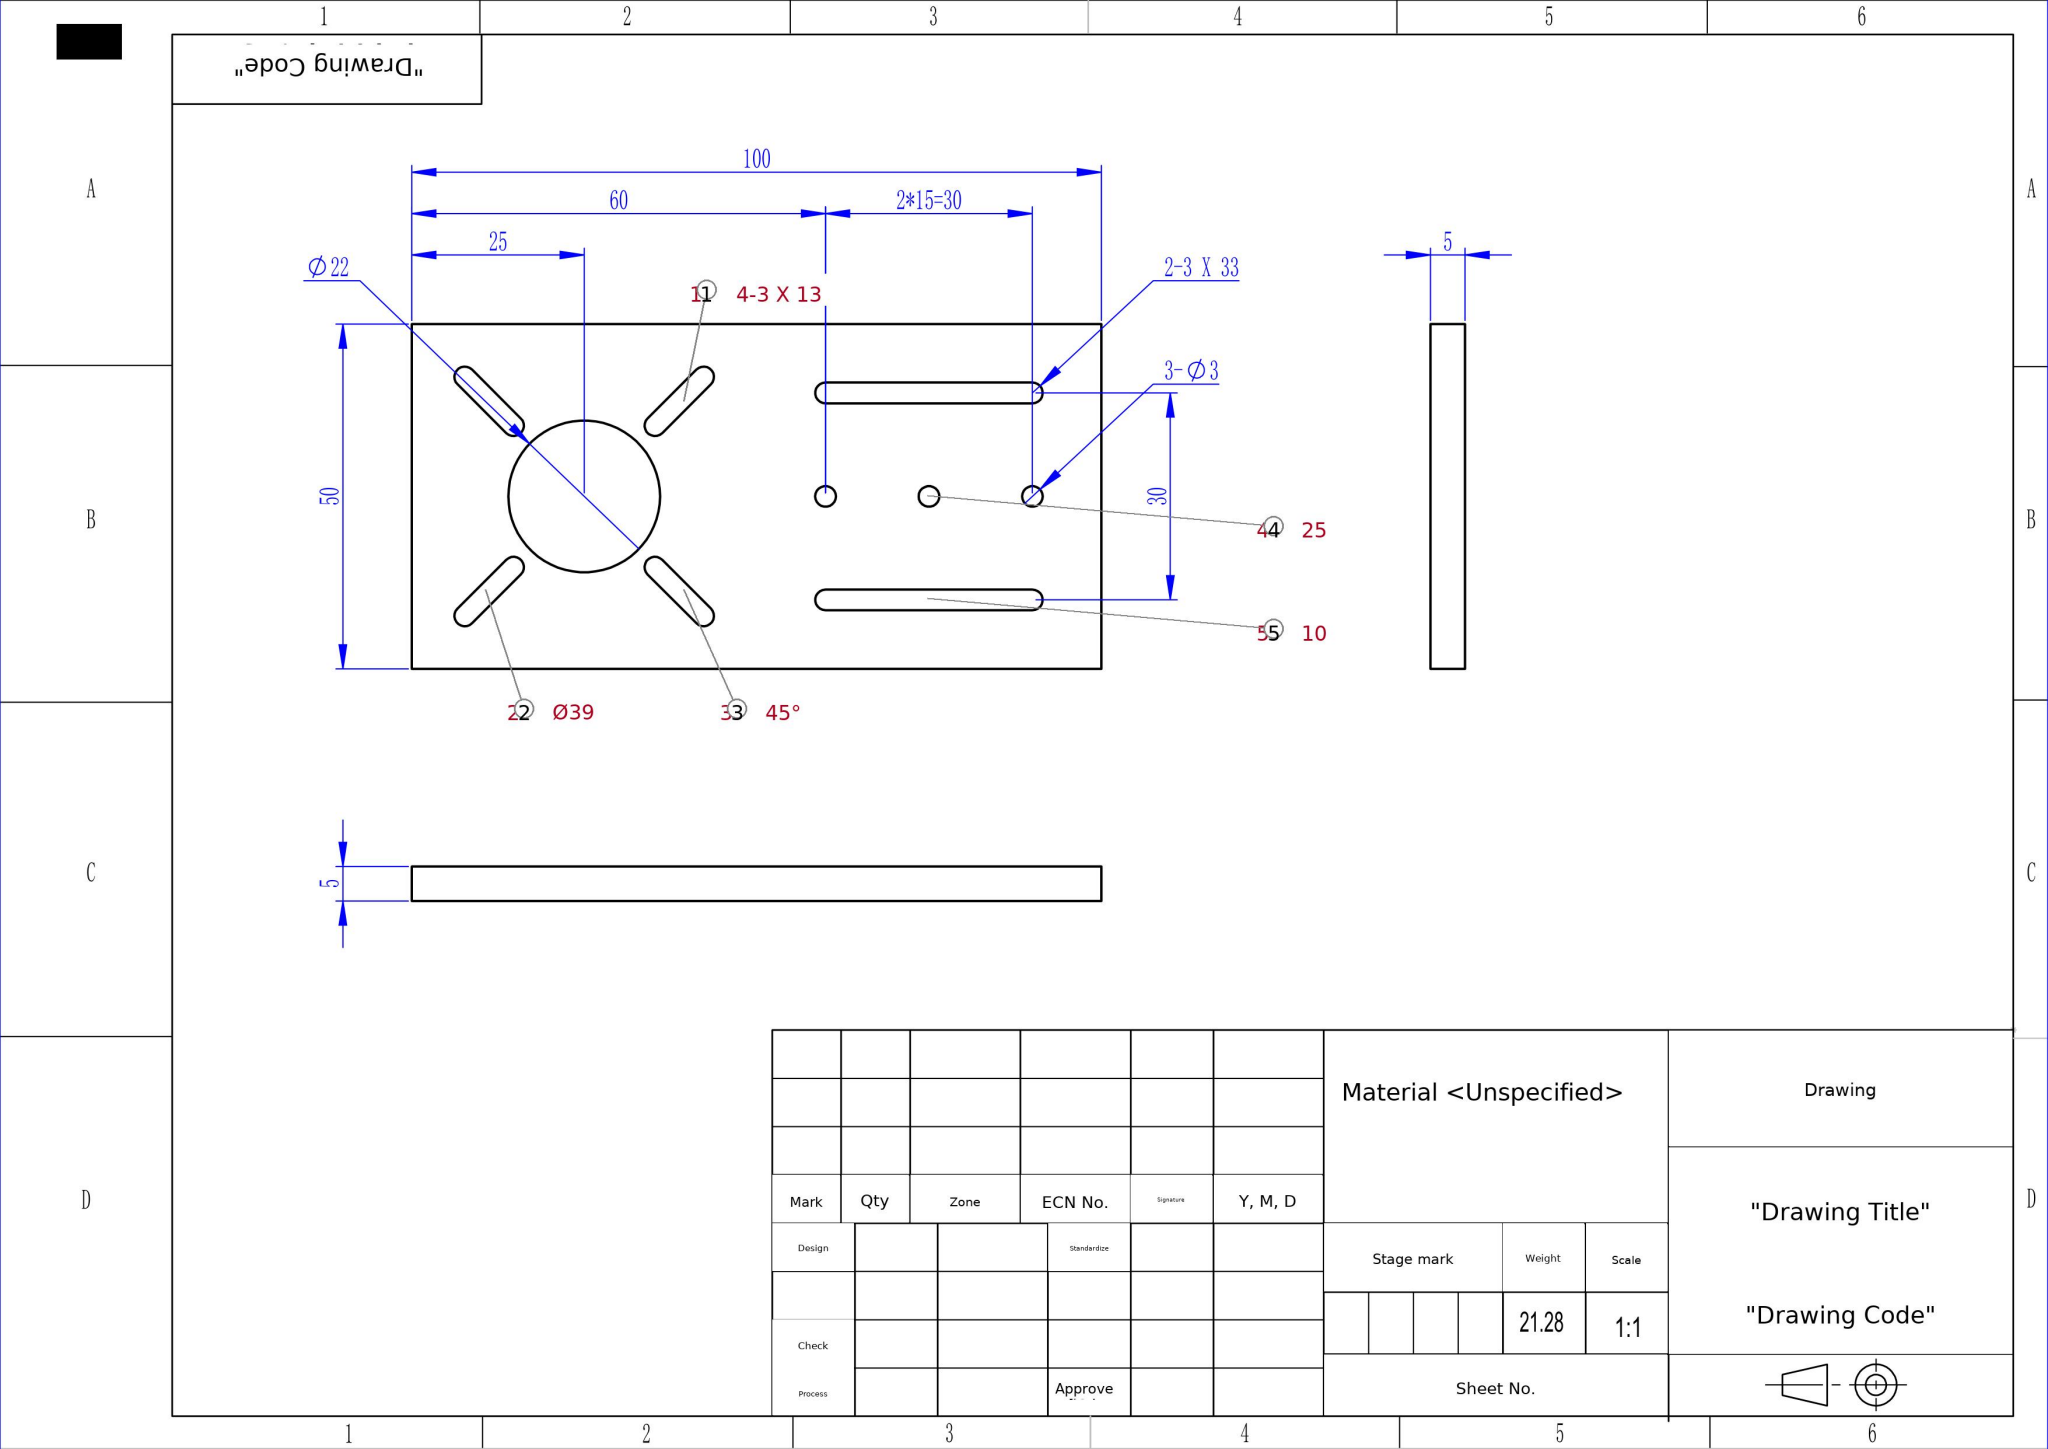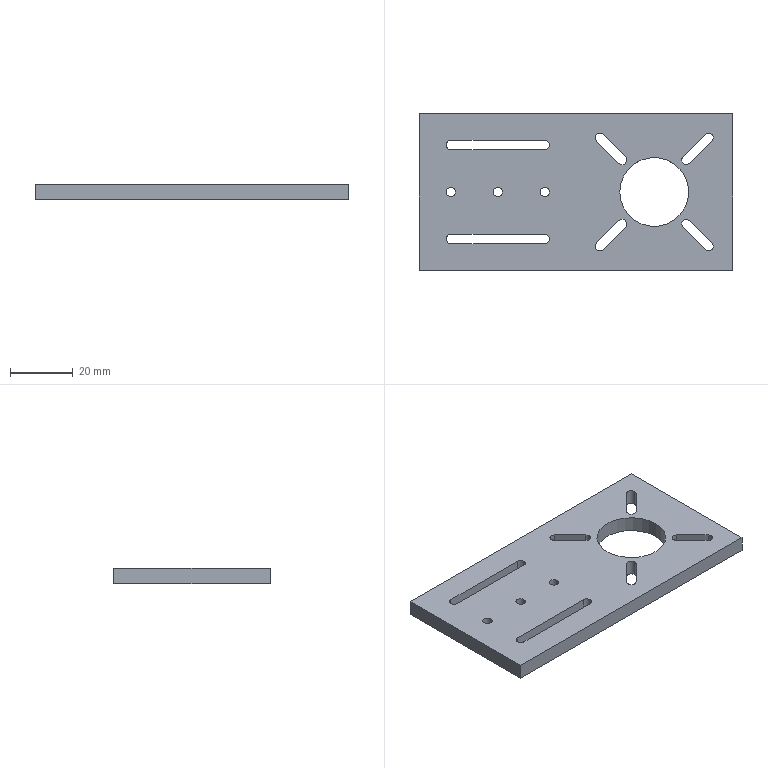Part | SolidWorks | mm | 1 solid | 44 faces | box 100 x 50 x 5 mm | volume 21281 mm3 | cylinder 26 | plane 18 | commonest cylinder face diameters 3 x24 22 x2
build123d program:
from build123d import *

# Parameters (mm, degrees)
BOSS_EXTRUDE1_DEPTH = 5


with BuildPart() as part:
    # Sketch1 → Boss-Extrude1 (new body)
    # profile 1 of 11: a face of its own
    with BuildSketch(Plane.XY):
        with BuildLine():
            Line((-8.5, 0), (0, 0))
            Line((0, 0), (0, 25))
            Line((0, 25), (-41.5, 25))
            Line((-41.5, 25), (-41.5, 15))
            Line((-41.5, 15), (-41.5, 0))
            ThreePointArc((-41.5, 0), (-40, 1.5), (-38.5, 0))
            Line((-38.5, 0), (-26.5, 0))
            ThreePointArc((-26.5, 0), (-25, 1.5), (-23.5, 0))
            Line((-23.5, 0), (-11.5, 0))
            ThreePointArc((-11.5, 0), (-10, 1.5), (-8.5, 0))
        make_face()
        with BuildLine():
            ThreePointArc((-40, 13.5), (-41.061, 13.939), (-41.5, 15))
            ThreePointArc((-41.5, 15), (-41.061, 16.061), (-40, 16.5))
            Line((-40, 16.5), (-10, 16.5))
            ThreePointArc((-10, 16.5), (-8.5, 15), (-10, 13.5))
            Line((-10, 13.5), (-40, 13.5))
        make_face(mode=Mode.SUBTRACT)
    # profile 2 of 11: a face of its own
    with BuildSketch(Plane.XY):
        Polygon((-41.5, 15), (-41.5, 25), (-50, 25), (-50, 0), (-41.5, 0), align=None)
    # profile 3 of 11: a face of its own
    with BuildSketch(Plane.XY):
        with BuildLine():
            Line((0, -25), (0, 0))
            Line((0, 0), (-8.5, 0))
            ThreePointArc((-8.5, 0), (-10, -1.5), (-11.5, 0))
            Line((-11.5, 0), (-23.5, 0))
            ThreePointArc((-23.5, 0), (-25, -1.5), (-26.5, 0))
            Line((-26.5, 0), (-38.5, 0))
            ThreePointArc((-38.5, 0), (-40, -1.5), (-41.5, 0))
            Line((-41.5, 0), (-50, 0))
            Line((-50, 0), (-50, -25))
            Line((-50, -25), (0, -25))
        make_face()
        with BuildLine():
            Line((-10, -16.5), (-40, -16.5))
            ThreePointArc((-40, -16.5), (-41.5, -15), (-40, -13.5))
            Line((-40, -13.5), (-10, -13.5))
            ThreePointArc((-10, -13.5), (-8.5, -15), (-10, -16.5))
        make_face(mode=Mode.SUBTRACT)
    # profile 4 of 11: a face of its own
    with BuildSketch(Plane.XY):
        with BuildLine():
            Line((0, 0), (14, 0))
            ThreePointArc((14, 0), (14.837, 4.21), (17.222, 7.778))
            Line((17.222, 7.778), (15.808, 9.192))
            ThreePointArc((15.808, 9.192), (14.747, 8.753), (13.686, 9.192))
            Line((13.686, 9.192), (6.615, 16.263))
            ThreePointArc((6.615, 16.263), (6.176, 17.324), (6.615, 18.385))
            Line((6.615, 18.385), (0, 25))
            Line((0, 25), (0, 0))
        make_face()
    # profile 5 of 11: a face of its own
    with BuildSketch(Plane.XY):
        with BuildLine():
            Line((15.808, 9.192), (17.222, 7.778))
            ThreePointArc((17.222, 7.778), (20.79, 10.163), (25, 11))
            Line((25, 11), (25, 25))
            Line((25, 25), (0, 25))
            Line((0, 25), (6.615, 18.385))
            ThreePointArc((6.615, 18.385), (7.676, 18.824), (8.737, 18.385))
            Line((8.737, 18.385), (15.808, 11.314))
            ThreePointArc((15.808, 11.314), (16.247, 10.253), (15.808, 9.192))
        make_face()
    # profile 6 of 11: a face of its own
    with BuildSketch(Plane.XY):
        with BuildLine():
            ThreePointArc((25, 11), (29.21, 10.163), (32.778, 7.778))
            Line((32.778, 7.778), (34.192, 9.192))
            ThreePointArc((34.192, 9.192), (33.753, 10.253), (34.192, 11.314))
            Line((34.192, 11.314), (41.263, 18.385))
            ThreePointArc((41.263, 18.385), (42.324, 18.824), (43.385, 18.385))
            Line((43.385, 18.385), (50, 25))
            Line((50, 25), (25, 25))
            Line((25, 25), (25, 11))
        make_face()
    # profile 7 of 11: a face of its own
    with BuildSketch(Plane.XY):
        with BuildLine():
            ThreePointArc((32.778, 7.778), (35.163, 4.21), (36, 0))
            Line((36, 0), (50, 0))
            Line((50, 0), (50, 25))
            Line((50, 25), (43.385, 18.385))
            ThreePointArc((43.385, 18.385), (43.824, 17.324), (43.385, 16.263))
            Line((43.385, 16.263), (36.314, 9.192))
            ThreePointArc((36.314, 9.192), (35.253, 8.753), (34.192, 9.192))
            Line((34.192, 9.192), (32.778, 7.778))
        make_face()
    # profile 8 of 11: a face of its own
    with BuildSketch(Plane.XY):
        with BuildLine():
            Line((50, 0), (36, 0))
            ThreePointArc((36, 0), (35.163, -4.21), (32.778, -7.778))
            Line((32.778, -7.778), (34.192, -9.192))
            ThreePointArc((34.192, -9.192), (35.253, -8.753), (36.314, -9.192))
            Line((36.314, -9.192), (43.385, -16.263))
            ThreePointArc((43.385, -16.263), (43.824, -17.324), (43.385, -18.385))
            Line((43.385, -18.385), (50, -25))
            Line((50, -25), (50, 0))
        make_face()
    # profile 9 of 11: a face of its own
    with BuildSketch(Plane.XY):
        with BuildLine():
            Line((34.192, -9.192), (32.778, -7.778))
            ThreePointArc((32.778, -7.778), (29.21, -10.163), (25, -11))
            Line((25, -11), (25, -25))
            Line((25, -25), (50, -25))
            Line((50, -25), (43.385, -18.385))
            ThreePointArc((43.385, -18.385), (42.324, -18.824), (41.263, -18.385))
            Line((41.263, -18.385), (34.192, -11.314))
            ThreePointArc((34.192, -11.314), (33.753, -10.253), (34.192, -9.192))
        make_face()
    # profile 10 of 11: a face of its own
    with BuildSketch(Plane.XY):
        with BuildLine():
            ThreePointArc((25, -11), (20.79, -10.163), (17.222, -7.778))
            Line((17.222, -7.778), (15.808, -9.192))
            ThreePointArc((15.808, -9.192), (16.247, -10.253), (15.808, -11.314))
            Line((15.808, -11.314), (8.737, -18.385))
            ThreePointArc((8.737, -18.385), (7.676, -18.824), (6.615, -18.385))
            Line((6.615, -18.385), (0, -25))
            Line((0, -25), (25, -25))
            Line((25, -25), (25, -11))
        make_face()
    # profile 11 of 11: a face of its own
    with BuildSketch(Plane.XY):
        with BuildLine():
            ThreePointArc((17.222, -7.778), (14.837, -4.21), (14, 0))
            Line((14, 0), (0, 0))
            Line((0, 0), (0, -25))
            Line((0, -25), (6.615, -18.385))
            ThreePointArc((6.615, -18.385), (6.176, -17.324), (6.615, -16.263))
            Line((6.615, -16.263), (13.686, -9.192))
            ThreePointArc((13.686, -9.192), (14.747, -8.753), (15.808, -9.192))
            Line((15.808, -9.192), (17.222, -7.778))
        make_face()
    extrude(amount=BOSS_EXTRUDE1_DEPTH)


solid = part.part